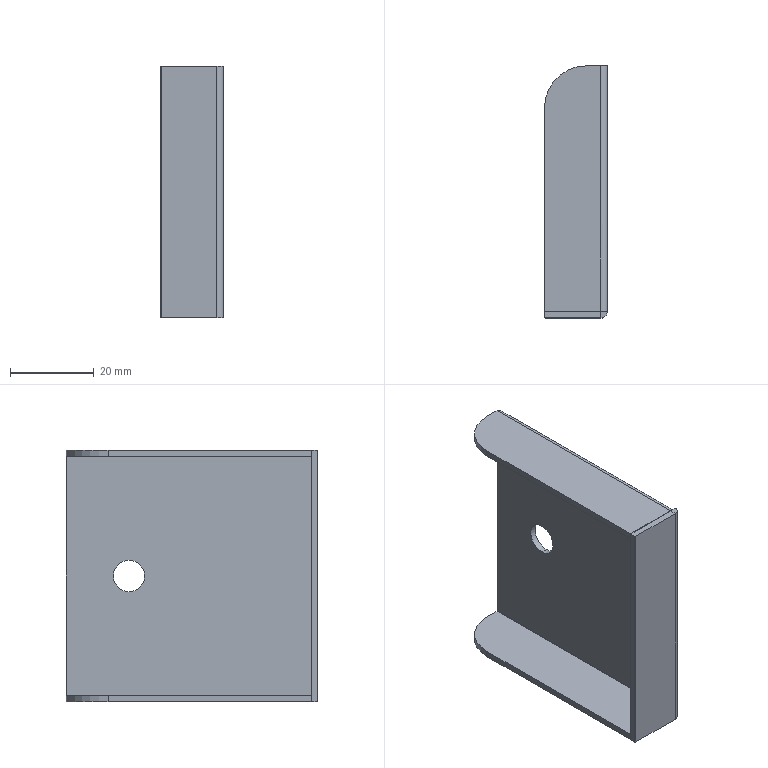Component | SolidWorks | BottomPlateWelding-2_AxisFixingPlate-2 | 1 solid | 37 faces | box 15 x 60 x 60 mm | volume 8752 mm3 | plane 27 | cylinder 10 | commonest cylinder face diameters 0.2 x3 3.2 x3 7.5 x2 20 x2
STEP:
#1=CARTESIAN_POINT('',(-9.252,0.7874,15.128));
#2=VERTEX_POINT('',#1);
#3=CARTESIAN_POINT('',(-9.252,0.7874,14.833));
#4=VERTEX_POINT('',#3);
#5=CARTESIAN_POINT('',(-9.252,0.7874,14.98));
#6=DIRECTION('',(1.,0.,-0.));
#7=DIRECTION('',(0.,0.,1.));
#8=AXIS2_PLACEMENT_3D('',#5,#6,#7);
#9=CIRCLE('',#8,0.1476);
#10=EDGE_CURVE('',#2,#4,#9,.T.);
#11=ORIENTED_EDGE('',*,*,#10,.F.);
#12=CARTESIAN_POINT('',(-9.193,0.7874,15.128));
#13=VERTEX_POINT('',#12);
#14=CARTESIAN_POINT('',(-9.67,0.7874,15.128));
#15=DIRECTION('',(1.,0.,-0.));
#16=VECTOR('',#15,39.37);
#17=LINE('',#14,#16);
#18=EDGE_CURVE('',#2,#13,#17,.T.);
#19=ORIENTED_EDGE('',*,*,#18,.T.);
#20=CARTESIAN_POINT('',(-9.193,0.7874,14.833));
#21=VERTEX_POINT('',#20);
#22=CARTESIAN_POINT('',(-9.193,0.7874,14.98));
#23=DIRECTION('',(1.,0.,-0.));
#24=DIRECTION('',(0.,-0.,-1.));
#25=AXIS2_PLACEMENT_3D('',#22,#23,#24);
#26=CIRCLE('',#25,0.1476);
#27=EDGE_CURVE('',#13,#21,#26,.T.);
#28=ORIENTED_EDGE('',*,*,#27,.T.);
#29=CARTESIAN_POINT('',(-9.67,0.7874,14.833));
#30=DIRECTION('',(1.,0.,-0.));
#31=VECTOR('',#30,39.37);
#32=LINE('',#29,#31);
#33=EDGE_CURVE('',#4,#21,#32,.T.);
#34=ORIENTED_EDGE('',*,*,#33,.F.);
#35=EDGE_LOOP('',(#11,#19,#28,#34));
#36=FACE_OUTER_BOUND('',#35,.T.);
#37=CARTESIAN_POINT('',(-9.67,0.7874,14.98));
#38=DIRECTION('',(1.,0.,-0.));
#39=DIRECTION('',(0.,-0.,-1.));
#40=AXIS2_PLACEMENT_3D('',#37,#38,#39);
#41=CYLINDRICAL_SURFACE('',#40,0.1476);
#42=ADVANCED_FACE('',(#36),#41,.F.);
#43=CARTESIAN_POINT('',(-9.193,-0.9213,16.161));
#44=VERTEX_POINT('',#43);
#45=CARTESIAN_POINT('',(-9.193,-0.9213,16.098));
#46=VERTEX_POINT('',#45);
#47=CARTESIAN_POINT('',(-9.193,-0.9213,13.799));
#48=DIRECTION('',(-0.,-0.,-1.));
#49=VECTOR('',#48,39.37);
#50=LINE('',#47,#49);
#51=EDGE_CURVE('',#44,#46,#50,.T.);
#52=ORIENTED_EDGE('',*,*,#51,.T.);
#53=CARTESIAN_POINT('',(-9.252,-0.9213,16.161));
#54=VERTEX_POINT('',#53);
#55=CARTESIAN_POINT('',(-9.256,-0.9213,16.098));
#56=DIRECTION('',(0.,-1.,0.));
#57=DIRECTION('',(0.,-0.,-1.));
#58=AXIS2_PLACEMENT_3D('',#55,#56,#57);
#59=CIRCLE('',#58,0.06299);
#60=EDGE_CURVE('',#46,#54,#59,.T.);
#61=ORIENTED_EDGE('',*,*,#60,.T.);
#62=CARTESIAN_POINT('',(-9.252,-0.9213,16.161));
#63=VERTEX_POINT('',#62);
#64=CARTESIAN_POINT('',(-9.252,-0.9213,16.098));
#65=DIRECTION('',(0.,0.,1.));
#66=VECTOR('',#65,39.37);
#67=LINE('',#64,#66);
#68=EDGE_CURVE('',#54,#63,#67,.T.);
#69=ORIENTED_EDGE('',*,*,#68,.T.);
#70=CARTESIAN_POINT('',(-9.252,-0.9213,16.161));
#71=DIRECTION('',(1.,-0.,-0.));
#72=VECTOR('',#71,39.37);
#73=LINE('',#70,#72);
#74=EDGE_CURVE('',#63,#44,#73,.T.);
#75=ORIENTED_EDGE('',*,*,#74,.T.);
#76=EDGE_LOOP('',(#52,#61,#69,#75));
#77=FACE_OUTER_BOUND('',#76,.T.);
#78=CARTESIAN_POINT('',(-9.252,-0.9213,16.098));
#79=DIRECTION('',(-0.,1.,-0.));
#80=DIRECTION('',(-0.,-0.,-1.));
#81=AXIS2_PLACEMENT_3D('',#78,#79,#80);
#82=PLANE('',#81);
#83=ADVANCED_FACE('',(#77),#82,.T.);
#84=CARTESIAN_POINT('',(-9.252,0.7874,14.98));
#85=DIRECTION('',(1.,0.,-0.));
#86=DIRECTION('',(0.,0.,1.));
#87=AXIS2_PLACEMENT_3D('',#84,#85,#86);
#88=CIRCLE('',#87,0.1476);
#89=EDGE_CURVE('',#4,#2,#88,.T.);
#90=ORIENTED_EDGE('',*,*,#89,.T.);
#91=ORIENTED_EDGE('',*,*,#10,.T.);
#92=EDGE_LOOP('',(#90,#91));
#93=FACE_BOUND('',#92,.T.);
#94=CARTESIAN_POINT('',(-9.252,-0.9213,13.862));
#95=VERTEX_POINT('',#94);
#96=CARTESIAN_POINT('',(-9.252,-0.9213,16.098));
#97=VERTEX_POINT('',#96);
#98=CARTESIAN_POINT('',(-9.252,-0.9213,13.799));
#99=DIRECTION('',(0.,0.,1.));
#100=VECTOR('',#99,39.37);
#101=LINE('',#98,#100);
#102=EDGE_CURVE('',#95,#97,#101,.T.);
#103=ORIENTED_EDGE('',*,*,#102,.T.);
#104=CARTESIAN_POINT('',(-9.252,1.378,16.098));
#105=VERTEX_POINT('',#104);
#106=CARTESIAN_POINT('',(-9.252,1.378,16.098));
#107=DIRECTION('',(0.,-1.,0.));
#108=VECTOR('',#107,39.37);
#109=LINE('',#106,#108);
#110=EDGE_CURVE('',#105,#97,#109,.T.);
#111=ORIENTED_EDGE('',*,*,#110,.F.);
#112=CARTESIAN_POINT('',(-9.252,1.378,13.862));
#113=VERTEX_POINT('',#112);
#114=CARTESIAN_POINT('',(-9.252,1.378,13.799));
#115=DIRECTION('',(0.,0.,1.));
#116=VECTOR('',#115,39.37);
#117=LINE('',#114,#116);
#118=EDGE_CURVE('',#113,#105,#117,.T.);
#119=ORIENTED_EDGE('',*,*,#118,.F.);
#120=CARTESIAN_POINT('',(-9.252,-0.9213,13.862));
#121=DIRECTION('',(-0.,1.,-0.));
#122=VECTOR('',#121,39.37);
#123=LINE('',#120,#122);
#124=EDGE_CURVE('',#95,#113,#123,.T.);
#125=ORIENTED_EDGE('',*,*,#124,.F.);
#126=EDGE_LOOP('',(#103,#111,#119,#125));
#127=FACE_OUTER_BOUND('',#126,.T.);
#128=CARTESIAN_POINT('',(-9.252,1.378,13.799));
#129=DIRECTION('',(-1.,-0.,0.));
#130=DIRECTION('',(0.,0.,1.));
#131=AXIS2_PLACEMENT_3D('',#128,#129,#130);
#132=PLANE('',#131);
#133=ADVANCED_FACE('',(#93,#127),#132,.T.);
#134=CARTESIAN_POINT('',(-9.193,0.7874,14.98));
#135=DIRECTION('',(1.,0.,-0.));
#136=DIRECTION('',(0.,-0.,-1.));
#137=AXIS2_PLACEMENT_3D('',#134,#135,#136);
#138=CIRCLE('',#137,0.1476);
#139=EDGE_CURVE('',#21,#13,#138,.T.);
#140=ORIENTED_EDGE('',*,*,#139,.F.);
#141=ORIENTED_EDGE('',*,*,#27,.F.);
#142=EDGE_LOOP('',(#140,#141));
#143=FACE_BOUND('',#142,.T.);
#144=CARTESIAN_POINT('',(-9.193,1.378,16.098));
#145=VERTEX_POINT('',#144);
#146=CARTESIAN_POINT('',(-9.193,1.378,16.098));
#147=DIRECTION('',(0.,-1.,0.));
#148=VECTOR('',#147,39.37);
#149=LINE('',#146,#148);
#150=EDGE_CURVE('',#145,#46,#149,.T.);
#151=ORIENTED_EDGE('',*,*,#150,.T.);
#152=CARTESIAN_POINT('',(-9.193,-0.9213,13.862));
#153=VERTEX_POINT('',#152);
#154=CARTESIAN_POINT('',(-9.193,-0.9213,13.799));
#155=DIRECTION('',(0.,0.,1.));
#156=VECTOR('',#155,39.37);
#157=LINE('',#154,#156);
#158=EDGE_CURVE('',#153,#46,#157,.T.);
#159=ORIENTED_EDGE('',*,*,#158,.F.);
#160=CARTESIAN_POINT('',(-9.193,1.378,13.862));
#161=VERTEX_POINT('',#160);
#162=CARTESIAN_POINT('',(-9.193,-0.9213,13.862));
#163=DIRECTION('',(-0.,1.,-0.));
#164=VECTOR('',#163,39.37);
#165=LINE('',#162,#164);
#166=EDGE_CURVE('',#153,#161,#165,.T.);
#167=ORIENTED_EDGE('',*,*,#166,.T.);
#168=CARTESIAN_POINT('',(-9.193,1.378,13.799));
#169=DIRECTION('',(0.,0.,1.));
#170=VECTOR('',#169,39.37);
#171=LINE('',#168,#170);
#172=EDGE_CURVE('',#161,#145,#171,.T.);
#173=ORIENTED_EDGE('',*,*,#172,.T.);
#174=EDGE_LOOP('',(#151,#159,#167,#173));
#175=FACE_OUTER_BOUND('',#174,.T.);
#176=CARTESIAN_POINT('',(-9.193,1.378,13.799));
#177=DIRECTION('',(-1.,-0.,0.));
#178=DIRECTION('',(0.,0.,1.));
#179=AXIS2_PLACEMENT_3D('',#176,#177,#178);
#180=PLANE('',#179);
#181=ADVANCED_FACE('',(#143,#175),#180,.F.);
#182=ORIENTED_EDGE('',*,*,#118,.T.);
#183=CARTESIAN_POINT('',(-9.252,1.378,16.098));
#184=DIRECTION('',(1.,0.,-0.));
#185=VECTOR('',#184,39.37);
#186=LINE('',#183,#185);
#187=EDGE_CURVE('',#105,#145,#186,.T.);
#188=ORIENTED_EDGE('',*,*,#187,.T.);
#189=ORIENTED_EDGE('',*,*,#172,.F.);
#190=CARTESIAN_POINT('',(-9.252,1.378,13.862));
#191=DIRECTION('',(1.,0.,-0.));
#192=VECTOR('',#191,39.37);
#193=LINE('',#190,#192);
#194=EDGE_CURVE('',#113,#161,#193,.T.);
#195=ORIENTED_EDGE('',*,*,#194,.F.);
#196=EDGE_LOOP('',(#182,#188,#189,#195));
#197=FACE_OUTER_BOUND('',#196,.T.);
#198=CARTESIAN_POINT('',(-9.193,1.378,13.799));
#199=DIRECTION('',(-0.,1.,-0.));
#200=DIRECTION('',(-0.,-0.,-1.));
#201=AXIS2_PLACEMENT_3D('',#198,#199,#200);
#202=PLANE('',#201);
#203=ADVANCED_FACE('',(#197),#202,.T.);
#204=CARTESIAN_POINT('',(-9.252,-0.9213,13.799));
#205=VERTEX_POINT('',#204);
#206=CARTESIAN_POINT('',(-9.252,-0.9213,13.799));
#207=VERTEX_POINT('',#206);
#208=CARTESIAN_POINT('',(-9.252,-0.9213,13.799));
#209=DIRECTION('',(0.,0.,1.));
#210=VECTOR('',#209,39.37);
#211=LINE('',#208,#210);
#212=EDGE_CURVE('',#205,#207,#211,.T.);
#213=ORIENTED_EDGE('',*,*,#212,.T.);
#214=CARTESIAN_POINT('',(-9.256,-0.9213,13.862));
#215=DIRECTION('',(0.,-1.,0.));
#216=DIRECTION('',(0.,0.,1.));
#217=AXIS2_PLACEMENT_3D('',#214,#215,#216);
#218=CIRCLE('',#217,0.06299);
#219=EDGE_CURVE('',#207,#153,#218,.T.);
#220=ORIENTED_EDGE('',*,*,#219,.T.);
#221=CARTESIAN_POINT('',(-9.193,-0.9213,13.799));
#222=VERTEX_POINT('',#221);
#223=CARTESIAN_POINT('',(-9.193,-0.9213,13.799));
#224=DIRECTION('',(0.,0.,1.));
#225=VECTOR('',#224,39.37);
#226=LINE('',#223,#225);
#227=EDGE_CURVE('',#222,#153,#226,.T.);
#228=ORIENTED_EDGE('',*,*,#227,.F.);
#229=CARTESIAN_POINT('',(-9.193,-0.9213,13.799));
#230=DIRECTION('',(-1.,0.,0.));
#231=VECTOR('',#230,39.37);
#232=LINE('',#229,#231);
#233=EDGE_CURVE('',#222,#205,#232,.T.);
#234=ORIENTED_EDGE('',*,*,#233,.T.);
#235=EDGE_LOOP('',(#213,#220,#228,#234));
#236=FACE_OUTER_BOUND('',#235,.T.);
#237=CARTESIAN_POINT('',(-9.252,-0.9213,13.799));
#238=DIRECTION('',(-0.,1.,-0.));
#239=DIRECTION('',(-0.,-0.,-1.));
#240=AXIS2_PLACEMENT_3D('',#237,#238,#239);
#241=PLANE('',#240);
#242=ADVANCED_FACE('',(#236),#241,.T.);
#243=ORIENTED_EDGE('',*,*,#233,.F.);
#244=CARTESIAN_POINT('',(-9.256,-0.9843,13.799));
#245=VERTEX_POINT('',#244);
#246=CARTESIAN_POINT('',(-9.256,-0.9213,13.799));
#247=DIRECTION('',(-0.,-0.,-1.));
#248=DIRECTION('',(1.,0.,0.));
#249=AXIS2_PLACEMENT_3D('',#246,#247,#248);
#250=CIRCLE('',#249,0.06299);
#251=EDGE_CURVE('',#222,#245,#250,.T.);
#252=ORIENTED_EDGE('',*,*,#251,.T.);
#253=CARTESIAN_POINT('',(-9.256,-0.9252,13.799));
#254=VERTEX_POINT('',#253);
#255=CARTESIAN_POINT('',(-9.256,-0.9252,13.799));
#256=DIRECTION('',(0.,-1.,0.));
#257=VECTOR('',#256,39.37);
#258=LINE('',#255,#257);
#259=EDGE_CURVE('',#254,#245,#258,.T.);
#260=ORIENTED_EDGE('',*,*,#259,.F.);
#261=CARTESIAN_POINT('',(-9.256,-0.9213,13.799));
#262=DIRECTION('',(-0.,-0.,-1.));
#263=DIRECTION('',(-1.,0.,0.));
#264=AXIS2_PLACEMENT_3D('',#261,#262,#263);
#265=CIRCLE('',#264,0.003937);
#266=EDGE_CURVE('',#205,#254,#265,.T.);
#267=ORIENTED_EDGE('',*,*,#266,.F.);
#268=EDGE_LOOP('',(#243,#252,#260,#267));
#269=FACE_OUTER_BOUND('',#268,.T.);
#270=CARTESIAN_POINT('',(-9.193,-0.9213,13.799));
#271=DIRECTION('',(-0.,-0.,-1.));
#272=DIRECTION('',(-1.,-0.,0.));
#273=AXIS2_PLACEMENT_3D('',#270,#271,#272);
#274=PLANE('',#273);
#275=ADVANCED_FACE('',(#269),#274,.T.);
#276=CARTESIAN_POINT('',(-9.256,-0.9843,16.161));
#277=VERTEX_POINT('',#276);
#278=CARTESIAN_POINT('',(-9.256,-0.9252,16.161));
#279=VERTEX_POINT('',#278);
#280=CARTESIAN_POINT('',(-9.256,-0.9843,16.161));
#281=DIRECTION('',(-0.,1.,-0.));
#282=VECTOR('',#281,39.37);
#283=LINE('',#280,#282);
#284=EDGE_CURVE('',#277,#279,#283,.T.);
#285=ORIENTED_EDGE('',*,*,#284,.F.);
#286=CARTESIAN_POINT('',(-9.256,-0.9213,16.161));
#287=DIRECTION('',(-0.,-0.,-1.));
#288=DIRECTION('',(1.,0.,0.));
#289=AXIS2_PLACEMENT_3D('',#286,#287,#288);
#290=CIRCLE('',#289,0.06299);
#291=EDGE_CURVE('',#44,#277,#290,.T.);
#292=ORIENTED_EDGE('',*,*,#291,.F.);
#293=ORIENTED_EDGE('',*,*,#74,.F.);
#294=CARTESIAN_POINT('',(-9.256,-0.9213,16.161));
#295=DIRECTION('',(-0.,-0.,-1.));
#296=DIRECTION('',(-1.,0.,0.));
#297=AXIS2_PLACEMENT_3D('',#294,#295,#296);
#298=CIRCLE('',#297,0.003937);
#299=EDGE_CURVE('',#63,#279,#298,.T.);
#300=ORIENTED_EDGE('',*,*,#299,.T.);
#301=EDGE_LOOP('',(#285,#292,#293,#300));
#302=FACE_OUTER_BOUND('',#301,.T.);
#303=CARTESIAN_POINT('',(-9.256,-0.9843,16.161));
#304=DIRECTION('',(0.,0.,1.));
#305=DIRECTION('',(1.,0.,-0.));
#306=AXIS2_PLACEMENT_3D('',#303,#304,#305);
#307=PLANE('',#306);
#308=ADVANCED_FACE('',(#302),#307,.T.);
#309=CARTESIAN_POINT('',(-9.783,-0.9252,16.161));
#310=VERTEX_POINT('',#309);
#311=CARTESIAN_POINT('',(-9.783,-0.9783,16.161));
#312=VERTEX_POINT('',#311);
#313=CARTESIAN_POINT('',(-9.783,-0.9252,16.161));
#314=DIRECTION('',(0.,-1.,0.));
#315=VECTOR('',#314,39.37);
#316=LINE('',#313,#315);
#317=EDGE_CURVE('',#310,#312,#316,.T.);
#318=ORIENTED_EDGE('',*,*,#317,.T.);
#319=CARTESIAN_POINT('',(-9.778,-0.9843,16.161));
#320=VERTEX_POINT('',#319);
#321=CARTESIAN_POINT('',(-9.546,-1.216,16.161));
#322=DIRECTION('',(0.7071,-0.7071,0.));
#323=VECTOR('',#322,39.37);
#324=LINE('',#321,#323);
#325=EDGE_CURVE('',#312,#320,#324,.T.);
#326=ORIENTED_EDGE('',*,*,#325,.T.);
#327=CARTESIAN_POINT('',(-9.193,-0.9843,16.161));
#328=DIRECTION('',(-1.,-0.,0.));
#329=VECTOR('',#328,39.37);
#330=LINE('',#327,#329);
#331=EDGE_CURVE('',#277,#320,#330,.T.);
#332=ORIENTED_EDGE('',*,*,#331,.F.);
#333=ORIENTED_EDGE('',*,*,#284,.T.);
#334=CARTESIAN_POINT('',(-9.193,-0.9252,16.161));
#335=DIRECTION('',(-1.,-0.,0.));
#336=VECTOR('',#335,39.37);
#337=LINE('',#334,#336);
#338=EDGE_CURVE('',#279,#310,#337,.T.);
#339=ORIENTED_EDGE('',*,*,#338,.T.);
#340=EDGE_LOOP('',(#318,#326,#332,#333,#339));
#341=FACE_OUTER_BOUND('',#340,.T.);
#342=CARTESIAN_POINT('',(-9.252,-0.9213,16.161));
#343=DIRECTION('',(0.,0.,1.));
#344=DIRECTION('',(1.,0.,-0.));
#345=AXIS2_PLACEMENT_3D('',#342,#343,#344);
#346=PLANE('',#345);
#347=ADVANCED_FACE('',(#341),#346,.T.);
#348=ORIENTED_EDGE('',*,*,#331,.T.);
#349=CARTESIAN_POINT('',(-9.778,-0.9843,13.799));
#350=VERTEX_POINT('',#349);
#351=CARTESIAN_POINT('',(-9.778,-0.9843,13.799));
#352=DIRECTION('',(-0.,-0.,-1.));
#353=VECTOR('',#352,39.37);
#354=LINE('',#351,#353);
#355=EDGE_CURVE('',#320,#350,#354,.T.);
#356=ORIENTED_EDGE('',*,*,#355,.T.);
#357=CARTESIAN_POINT('',(-9.193,-0.9843,13.799));
#358=DIRECTION('',(-1.,-0.,0.));
#359=VECTOR('',#358,39.37);
#360=LINE('',#357,#359);
#361=EDGE_CURVE('',#245,#350,#360,.T.);
#362=ORIENTED_EDGE('',*,*,#361,.F.);
#363=CARTESIAN_POINT('',(-9.256,-0.9843,13.799));
#364=DIRECTION('',(0.,0.,1.));
#365=VECTOR('',#364,39.37);
#366=LINE('',#363,#365);
#367=EDGE_CURVE('',#245,#277,#366,.T.);
#368=ORIENTED_EDGE('',*,*,#367,.T.);
#369=EDGE_LOOP('',(#348,#356,#362,#368));
#370=FACE_OUTER_BOUND('',#369,.T.);
#371=CARTESIAN_POINT('',(-9.193,-0.9843,13.799));
#372=DIRECTION('',(-0.,1.,-0.));
#373=DIRECTION('',(-0.,-0.,-1.));
#374=AXIS2_PLACEMENT_3D('',#371,#372,#373);
#375=PLANE('',#374);
#376=ADVANCED_FACE('',(#370),#375,.F.);
#377=CARTESIAN_POINT('',(-9.783,-0.9252,13.799));
#378=VERTEX_POINT('',#377);
#379=CARTESIAN_POINT('',(-9.783,-0.9783,13.799));
#380=VERTEX_POINT('',#379);
#381=CARTESIAN_POINT('',(-9.783,-0.9252,13.799));
#382=DIRECTION('',(0.,-1.,0.));
#383=VECTOR('',#382,39.37);
#384=LINE('',#381,#383);
#385=EDGE_CURVE('',#378,#380,#384,.T.);
#386=ORIENTED_EDGE('',*,*,#385,.T.);
#387=CARTESIAN_POINT('',(-9.783,-0.9783,16.161));
#388=DIRECTION('',(0.,0.,1.));
#389=VECTOR('',#388,39.37);
#390=LINE('',#387,#389);
#391=EDGE_CURVE('',#380,#312,#390,.T.);
#392=ORIENTED_EDGE('',*,*,#391,.T.);
#393=ORIENTED_EDGE('',*,*,#317,.F.);
#394=CARTESIAN_POINT('',(-9.783,-0.9252,13.799));
#395=DIRECTION('',(0.,0.,1.));
#396=VECTOR('',#395,39.37);
#397=LINE('',#394,#396);
#398=EDGE_CURVE('',#378,#310,#397,.T.);
#399=ORIENTED_EDGE('',*,*,#398,.F.);
#400=EDGE_LOOP('',(#386,#392,#393,#399));
#401=FACE_OUTER_BOUND('',#400,.T.);
#402=CARTESIAN_POINT('',(-9.783,-0.9252,13.799));
#403=DIRECTION('',(-1.,-0.,0.));
#404=DIRECTION('',(0.,0.,1.));
#405=AXIS2_PLACEMENT_3D('',#402,#403,#404);
#406=PLANE('',#405);
#407=ADVANCED_FACE('',(#401),#406,.T.);
#408=ORIENTED_EDGE('',*,*,#338,.F.);
#409=CARTESIAN_POINT('',(-9.256,-0.9252,13.799));
#410=DIRECTION('',(0.,0.,1.));
#411=VECTOR('',#410,39.37);
#412=LINE('',#409,#411);
#413=EDGE_CURVE('',#254,#279,#412,.T.);
#414=ORIENTED_EDGE('',*,*,#413,.F.);
#415=CARTESIAN_POINT('',(-9.193,-0.9252,13.799));
#416=DIRECTION('',(-1.,-0.,0.));
#417=VECTOR('',#416,39.37);
#418=LINE('',#415,#417);
#419=EDGE_CURVE('',#254,#378,#418,.T.);
#420=ORIENTED_EDGE('',*,*,#419,.T.);
#421=ORIENTED_EDGE('',*,*,#398,.T.);
#422=EDGE_LOOP('',(#408,#414,#420,#421));
#423=FACE_OUTER_BOUND('',#422,.T.);
#424=CARTESIAN_POINT('',(-9.193,-0.9252,13.799));
#425=DIRECTION('',(-0.,1.,-0.));
#426=DIRECTION('',(-0.,-0.,-1.));
#427=AXIS2_PLACEMENT_3D('',#424,#425,#426);
#428=PLANE('',#427);
#429=ADVANCED_FACE('',(#423),#428,.T.);
#430=ORIENTED_EDGE('',*,*,#299,.F.);
#431=ORIENTED_EDGE('',*,*,#68,.F.);
#432=CARTESIAN_POINT('',(-9.252,-0.9213,16.098));
#433=DIRECTION('',(0.,0.,1.));
#434=VECTOR('',#433,39.37);
#435=LINE('',#432,#434);
#436=EDGE_CURVE('',#97,#54,#435,.T.);
#437=ORIENTED_EDGE('',*,*,#436,.F.);
#438=ORIENTED_EDGE('',*,*,#102,.F.);
#439=CARTESIAN_POINT('',(-9.252,-0.9213,13.799));
#440=DIRECTION('',(0.,0.,1.));
#441=VECTOR('',#440,39.37);
#442=LINE('',#439,#441);
#443=EDGE_CURVE('',#207,#95,#442,.T.);
#444=ORIENTED_EDGE('',*,*,#443,.F.);
#445=ORIENTED_EDGE('',*,*,#212,.F.);
#446=ORIENTED_EDGE('',*,*,#266,.T.);
#447=ORIENTED_EDGE('',*,*,#413,.T.);
#448=EDGE_LOOP('',(#430,#431,#437,#438,#444,#445,#446,#447));
#449=FACE_OUTER_BOUND('',#448,.T.);
#450=CARTESIAN_POINT('',(-9.256,-0.9213,13.799));
#451=DIRECTION('',(0.,0.,1.));
#452=DIRECTION('',(1.,0.,0.));
#453=AXIS2_PLACEMENT_3D('',#450,#451,#452);
#454=CYLINDRICAL_SURFACE('',#453,0.003937);
#455=ADVANCED_FACE('',(#449),#454,.F.);
#456=ORIENTED_EDGE('',*,*,#291,.T.);
#457=ORIENTED_EDGE('',*,*,#367,.F.);
#458=ORIENTED_EDGE('',*,*,#251,.F.);
#459=ORIENTED_EDGE('',*,*,#227,.T.);
#460=ORIENTED_EDGE('',*,*,#158,.T.);
#461=ORIENTED_EDGE('',*,*,#51,.F.);
#462=EDGE_LOOP('',(#456,#457,#458,#459,#460,#461));
#463=FACE_OUTER_BOUND('',#462,.T.);
#464=CARTESIAN_POINT('',(-9.256,-0.9213,13.799));
#465=DIRECTION('',(0.,0.,1.));
#466=DIRECTION('',(1.,0.,0.));
#467=AXIS2_PLACEMENT_3D('',#464,#465,#466);
#468=CYLINDRICAL_SURFACE('',#467,0.06299);
#469=ADVANCED_FACE('',(#463),#468,.T.);
#470=ORIENTED_EDGE('',*,*,#361,.T.);
#471=CARTESIAN_POINT('',(-9.548,-1.214,13.799));
#472=DIRECTION('',(-0.7071,0.7071,-0.));
#473=VECTOR('',#472,39.37);
#474=LINE('',#471,#473);
#475=EDGE_CURVE('',#350,#380,#474,.T.);
#476=ORIENTED_EDGE('',*,*,#475,.T.);
#477=ORIENTED_EDGE('',*,*,#385,.F.);
#478=ORIENTED_EDGE('',*,*,#419,.F.);
#479=ORIENTED_EDGE('',*,*,#259,.T.);
#480=EDGE_LOOP('',(#470,#476,#477,#478,#479));
#481=FACE_OUTER_BOUND('',#480,.T.);
#482=CARTESIAN_POINT('',(-9.256,-0.9213,13.799));
#483=DIRECTION('',(-0.,-0.,-1.));
#484=DIRECTION('',(-1.,-0.,0.));
#485=AXIS2_PLACEMENT_3D('',#482,#483,#484);
#486=PLANE('',#485);
#487=ADVANCED_FACE('',(#481),#486,.T.);
#488=ORIENTED_EDGE('',*,*,#18,.F.);
#489=ORIENTED_EDGE('',*,*,#89,.F.);
#490=ORIENTED_EDGE('',*,*,#33,.T.);
#491=ORIENTED_EDGE('',*,*,#139,.T.);
#492=EDGE_LOOP('',(#488,#489,#490,#491));
#493=FACE_OUTER_BOUND('',#492,.T.);
#494=CARTESIAN_POINT('',(-9.67,0.7874,14.98));
#495=DIRECTION('',(1.,0.,-0.));
#496=DIRECTION('',(0.,-0.,-1.));
#497=AXIS2_PLACEMENT_3D('',#494,#495,#496);
#498=CYLINDRICAL_SURFACE('',#497,0.1476);
#499=ADVANCED_FACE('',(#493),#498,.F.);
#500=CARTESIAN_POINT('',(-9.256,1.378,13.858));
#501=VERTEX_POINT('',#500);
#502=CARTESIAN_POINT('',(-9.256,1.378,13.799));
#503=VERTEX_POINT('',#502);
#504=CARTESIAN_POINT('',(-9.256,1.378,13.799));
#505=DIRECTION('',(-0.,-0.,-1.));
#506=VECTOR('',#505,39.37);
#507=LINE('',#504,#506);
#508=EDGE_CURVE('',#501,#503,#507,.T.);
#509=ORIENTED_EDGE('',*,*,#508,.F.);
#510=CARTESIAN_POINT('',(-9.256,1.378,13.862));
#511=DIRECTION('',(-0.,1.,-0.));
#512=DIRECTION('',(0.,0.,1.));
#513=AXIS2_PLACEMENT_3D('',#510,#511,#512);
#514=CIRCLE('',#513,0.003937);
#515=EDGE_CURVE('',#113,#501,#514,.T.);
#516=ORIENTED_EDGE('',*,*,#515,.F.);
#517=ORIENTED_EDGE('',*,*,#194,.T.);
#518=CARTESIAN_POINT('',(-9.256,1.378,13.862));
#519=DIRECTION('',(-0.,1.,-0.));
#520=DIRECTION('',(0.,0.,1.));
#521=AXIS2_PLACEMENT_3D('',#518,#519,#520);
#522=CIRCLE('',#521,0.06299);
#523=EDGE_CURVE('',#161,#503,#522,.T.);
#524=ORIENTED_EDGE('',*,*,#523,.T.);
#525=EDGE_LOOP('',(#509,#516,#517,#524));
#526=FACE_OUTER_BOUND('',#525,.T.);
#527=CARTESIAN_POINT('',(-9.256,1.378,13.862));
#528=DIRECTION('',(-0.,1.,-0.));
#529=DIRECTION('',(-0.,-0.,-1.));
#530=AXIS2_PLACEMENT_3D('',#527,#528,#529);
#531=PLANE('',#530);
#532=ADVANCED_FACE('',(#526),#531,.T.);
#533=CARTESIAN_POINT('',(-9.256,-0.9213,13.799));
#534=VERTEX_POINT('',#533);
#535=CARTESIAN_POINT('',(-9.256,-0.9213,13.862));
#536=DIRECTION('',(0.,-1.,0.));
#537=DIRECTION('',(0.,0.,1.));
#538=AXIS2_PLACEMENT_3D('',#535,#536,#537);
#539=CIRCLE('',#538,0.06299);
#540=EDGE_CURVE('',#534,#207,#539,.T.);
#541=ORIENTED_EDGE('',*,*,#540,.T.);
#542=ORIENTED_EDGE('',*,*,#443,.T.);
#543=CARTESIAN_POINT('',(-9.256,-0.9213,13.858));
#544=VERTEX_POINT('',#543);
#545=CARTESIAN_POINT('',(-9.256,-0.9213,13.862));
#546=DIRECTION('',(0.,-1.,0.));
#547=DIRECTION('',(0.,0.,1.));
#548=AXIS2_PLACEMENT_3D('',#545,#546,#547);
#549=CIRCLE('',#548,0.003937);
#550=EDGE_CURVE('',#544,#95,#549,.T.);
#551=ORIENTED_EDGE('',*,*,#550,.F.);
#552=CARTESIAN_POINT('',(-9.256,-0.9213,13.858));
#553=DIRECTION('',(-0.,-0.,-1.));
#554=VECTOR('',#553,39.37);
#555=LINE('',#552,#554);
#556=EDGE_CURVE('',#544,#534,#555,.T.);
#557=ORIENTED_EDGE('',*,*,#556,.T.);
#558=EDGE_LOOP('',(#541,#542,#551,#557));
#559=FACE_OUTER_BOUND('',#558,.T.);
#560=CARTESIAN_POINT('',(-9.256,-0.9213,13.862));
#561=DIRECTION('',(-0.,1.,-0.));
#562=DIRECTION('',(-0.,-0.,-1.));
#563=AXIS2_PLACEMENT_3D('',#560,#561,#562);
#564=PLANE('',#563);
#565=ADVANCED_FACE('',(#559),#564,.F.);
#566=ORIENTED_EDGE('',*,*,#166,.F.);
#567=ORIENTED_EDGE('',*,*,#219,.F.);
#568=ORIENTED_EDGE('',*,*,#540,.F.);
#569=CARTESIAN_POINT('',(-9.256,-0.9843,13.799));
#570=DIRECTION('',(0.,-1.,0.));
#571=VECTOR('',#570,39.37);
#572=LINE('',#569,#571);
#573=EDGE_CURVE('',#503,#534,#572,.T.);
#574=ORIENTED_EDGE('',*,*,#573,.F.);
#575=ORIENTED_EDGE('',*,*,#523,.F.);
#576=EDGE_LOOP('',(#566,#567,#568,#574,#575));
#577=FACE_OUTER_BOUND('',#576,.T.);
#578=CARTESIAN_POINT('',(-9.256,-0.9213,13.862));
#579=DIRECTION('',(0.,-1.,0.));
#580=DIRECTION('',(0.,-0.,-1.));
#581=AXIS2_PLACEMENT_3D('',#578,#579,#580);
#582=CYLINDRICAL_SURFACE('',#581,0.06299);
#583=ADVANCED_FACE('',(#577),#582,.T.);
#584=ORIENTED_EDGE('',*,*,#124,.T.);
#585=ORIENTED_EDGE('',*,*,#515,.T.);
#586=CARTESIAN_POINT('',(-9.256,1.378,13.858));
#587=DIRECTION('',(0.,-1.,0.));
#588=VECTOR('',#587,39.37);
#589=LINE('',#586,#588);
#590=EDGE_CURVE('',#501,#544,#589,.T.);
#591=ORIENTED_EDGE('',*,*,#590,.T.);
#592=ORIENTED_EDGE('',*,*,#550,.T.);
#593=EDGE_LOOP('',(#584,#585,#591,#592));
#594=FACE_OUTER_BOUND('',#593,.T.);
#595=CARTESIAN_POINT('',(-9.256,-0.9213,13.862));
#596=DIRECTION('',(0.,-1.,0.));
#597=DIRECTION('',(0.,0.,-1.));
#598=AXIS2_PLACEMENT_3D('',#595,#596,#597);
#599=CYLINDRICAL_SURFACE('',#598,0.003937);
#600=ADVANCED_FACE('',(#594),#599,.F.);
#601=CARTESIAN_POINT('',(-9.39,1.378,13.799));
#602=VERTEX_POINT('',#601);
#603=CARTESIAN_POINT('',(-9.193,1.378,13.799));
#604=DIRECTION('',(1.,0.,0.));
#605=VECTOR('',#604,39.37);
#606=LINE('',#603,#605);
#607=EDGE_CURVE('',#602,#503,#606,.T.);
#608=ORIENTED_EDGE('',*,*,#607,.F.);
#609=CARTESIAN_POINT('',(-9.39,1.378,13.858));
#610=VERTEX_POINT('',#609);
#611=CARTESIAN_POINT('',(-9.39,1.378,13.799));
#612=DIRECTION('',(-0.,0.,1.));
#613=VECTOR('',#612,39.37);
#614=LINE('',#611,#613);
#615=EDGE_CURVE('',#602,#610,#614,.T.);
#616=ORIENTED_EDGE('',*,*,#615,.T.);
#617=CARTESIAN_POINT('',(-9.252,1.378,13.858));
#618=DIRECTION('',(1.,0.,0.));
#619=VECTOR('',#618,39.37);
#620=LINE('',#617,#619);
#621=EDGE_CURVE('',#610,#501,#620,.T.);
#622=ORIENTED_EDGE('',*,*,#621,.T.);
#623=ORIENTED_EDGE('',*,*,#508,.T.);
#624=EDGE_LOOP('',(#608,#616,#622,#623));
#625=FACE_OUTER_BOUND('',#624,.T.);
#626=CARTESIAN_POINT('',(-9.252,1.378,13.799));
#627=DIRECTION('',(0.,-1.,0.));
#628=DIRECTION('',(0.,0.,1.));
#629=AXIS2_PLACEMENT_3D('',#626,#627,#628);
#630=PLANE('',#629);
#631=ADVANCED_FACE('',(#625),#630,.F.);
#632=ORIENTED_EDGE('',*,*,#556,.F.);
#633=CARTESIAN_POINT('',(-9.783,-0.9213,13.858));
#634=VERTEX_POINT('',#633);
#635=CARTESIAN_POINT('',(-9.783,-0.9213,13.858));
#636=DIRECTION('',(-1.,-0.,-0.));
#637=VECTOR('',#636,39.37);
#638=LINE('',#635,#637);
#639=EDGE_CURVE('',#544,#634,#638,.T.);
#640=ORIENTED_EDGE('',*,*,#639,.T.);
#641=CARTESIAN_POINT('',(-9.783,-0.9213,13.799));
#642=VERTEX_POINT('',#641);
#643=CARTESIAN_POINT('',(-9.783,-0.9213,13.799));
#644=DIRECTION('',(-0.,0.,1.));
#645=VECTOR('',#644,39.37);
#646=LINE('',#643,#645);
#647=EDGE_CURVE('',#642,#634,#646,.T.);
#648=ORIENTED_EDGE('',*,*,#647,.F.);
#649=CARTESIAN_POINT('',(-9.193,-0.9213,13.799));
#650=DIRECTION('',(-1.,-0.,-0.));
#651=VECTOR('',#650,39.37);
#652=LINE('',#649,#651);
#653=EDGE_CURVE('',#534,#642,#652,.T.);
#654=ORIENTED_EDGE('',*,*,#653,.F.);
#655=EDGE_LOOP('',(#632,#640,#648,#654));
#656=FACE_OUTER_BOUND('',#655,.T.);
#657=CARTESIAN_POINT('',(-9.783,-0.9213,13.799));
#658=DIRECTION('',(-0.,1.,-0.));
#659=DIRECTION('',(-0.,-0.,-1.));
#660=AXIS2_PLACEMENT_3D('',#657,#658,#659);
#661=PLANE('',#660);
#662=ADVANCED_FACE('',(#656),#661,.F.);
#663=CARTESIAN_POINT('',(-9.783,0.9843,13.799));
#664=VERTEX_POINT('',#663);
#665=CARTESIAN_POINT('',(-9.783,-0.9843,13.799));
#666=DIRECTION('',(-0.,1.,-0.));
#667=VECTOR('',#666,39.37);
#668=LINE('',#665,#667);
#669=EDGE_CURVE('',#642,#664,#668,.T.);
#670=ORIENTED_EDGE('',*,*,#669,.T.);
#671=CARTESIAN_POINT('',(-9.39,0.9843,13.799));
#672=DIRECTION('',(0.,-0.,-1.));
#673=DIRECTION('',(-1.,0.,0.));
#674=AXIS2_PLACEMENT_3D('',#671,#672,#673);
#675=CIRCLE('',#674,0.3937);
#676=EDGE_CURVE('',#664,#602,#675,.T.);
#677=ORIENTED_EDGE('',*,*,#676,.T.);
#678=ORIENTED_EDGE('',*,*,#607,.T.);
#679=ORIENTED_EDGE('',*,*,#573,.T.);
#680=ORIENTED_EDGE('',*,*,#653,.T.);
#681=EDGE_LOOP('',(#670,#677,#678,#679,#680));
#682=FACE_OUTER_BOUND('',#681,.T.);
#683=CARTESIAN_POINT('',(-9.193,-0.9843,13.799));
#684=DIRECTION('',(0.,-0.,-1.));
#685=DIRECTION('',(-1.,-0.,-0.));
#686=AXIS2_PLACEMENT_3D('',#683,#684,#685);
#687=PLANE('',#686);
#688=ADVANCED_FACE('',(#682),#687,.T.);
#689=ORIENTED_EDGE('',*,*,#621,.F.);
#690=CARTESIAN_POINT('',(-9.783,0.9843,13.858));
#691=VERTEX_POINT('',#690);
#692=CARTESIAN_POINT('',(-9.39,0.9843,13.858));
#693=DIRECTION('',(-0.,0.,1.));
#694=DIRECTION('',(-1.,0.,0.));
#695=AXIS2_PLACEMENT_3D('',#692,#693,#694);
#696=CIRCLE('',#695,0.3937);
#697=EDGE_CURVE('',#610,#691,#696,.T.);
#698=ORIENTED_EDGE('',*,*,#697,.T.);
#699=CARTESIAN_POINT('',(-9.783,-0.9213,13.858));
#700=DIRECTION('',(-0.,1.,-0.));
#701=VECTOR('',#700,39.37);
#702=LINE('',#699,#701);
#703=EDGE_CURVE('',#634,#691,#702,.T.);
#704=ORIENTED_EDGE('',*,*,#703,.F.);
#705=ORIENTED_EDGE('',*,*,#639,.F.);
#706=ORIENTED_EDGE('',*,*,#590,.F.);
#707=EDGE_LOOP('',(#689,#698,#704,#705,#706));
#708=FACE_OUTER_BOUND('',#707,.T.);
#709=CARTESIAN_POINT('',(-9.193,-0.9843,13.858));
#710=DIRECTION('',(0.,-0.,-1.));
#711=DIRECTION('',(-1.,-0.,-0.));
#712=AXIS2_PLACEMENT_3D('',#709,#710,#711);
#713=PLANE('',#712);
#714=ADVANCED_FACE('',(#708),#713,.F.);
#715=ORIENTED_EDGE('',*,*,#703,.T.);
#716=CARTESIAN_POINT('',(-9.783,0.9843,13.799));
#717=DIRECTION('',(0.,-0.,-1.));
#718=VECTOR('',#717,39.37);
#719=LINE('',#716,#718);
#720=EDGE_CURVE('',#691,#664,#719,.T.);
#721=ORIENTED_EDGE('',*,*,#720,.T.);
#722=ORIENTED_EDGE('',*,*,#669,.F.);
#723=ORIENTED_EDGE('',*,*,#647,.T.);
#724=EDGE_LOOP('',(#715,#721,#722,#723));
#725=FACE_OUTER_BOUND('',#724,.T.);
#726=CARTESIAN_POINT('',(-9.783,-0.9213,13.799));
#727=DIRECTION('',(1.,0.,0.));
#728=DIRECTION('',(0.,-0.,-1.));
#729=AXIS2_PLACEMENT_3D('',#726,#727,#728);
#730=PLANE('',#729);
#731=ADVANCED_FACE('',(#725),#730,.F.);
#732=CARTESIAN_POINT('',(-9.256,-0.9213,16.102));
#733=VERTEX_POINT('',#732);
#734=CARTESIAN_POINT('',(-9.256,-0.9213,16.098));
#735=DIRECTION('',(0.,-1.,0.));
#736=DIRECTION('',(0.,0.,-1.));
#737=AXIS2_PLACEMENT_3D('',#734,#735,#736);
#738=CIRCLE('',#737,0.003937);
#739=EDGE_CURVE('',#97,#733,#738,.T.);
#740=ORIENTED_EDGE('',*,*,#739,.F.);
#741=ORIENTED_EDGE('',*,*,#436,.T.);
#742=CARTESIAN_POINT('',(-9.256,-0.9213,16.161));
#743=VERTEX_POINT('',#742);
#744=CARTESIAN_POINT('',(-9.256,-0.9213,16.098));
#745=DIRECTION('',(0.,-1.,0.));
#746=DIRECTION('',(0.,-0.,-1.));
#747=AXIS2_PLACEMENT_3D('',#744,#745,#746);
#748=CIRCLE('',#747,0.06299);
#749=EDGE_CURVE('',#54,#743,#748,.T.);
#750=ORIENTED_EDGE('',*,*,#749,.T.);
#751=CARTESIAN_POINT('',(-9.256,-0.9213,16.161));
#752=DIRECTION('',(0.,0.,1.));
#753=VECTOR('',#752,39.37);
#754=LINE('',#751,#753);
#755=EDGE_CURVE('',#733,#743,#754,.T.);
#756=ORIENTED_EDGE('',*,*,#755,.F.);
#757=EDGE_LOOP('',(#740,#741,#750,#756));
#758=FACE_OUTER_BOUND('',#757,.T.);
#759=CARTESIAN_POINT('',(-9.256,-0.9213,16.098));
#760=DIRECTION('',(0.,-1.,0.));
#761=DIRECTION('',(0.,0.,1.));
#762=AXIS2_PLACEMENT_3D('',#759,#760,#761);
#763=PLANE('',#762);
#764=ADVANCED_FACE('',(#758),#763,.T.);
#765=CARTESIAN_POINT('',(-9.256,1.378,16.102));
#766=VERTEX_POINT('',#765);
#767=CARTESIAN_POINT('',(-9.256,1.378,16.098));
#768=DIRECTION('',(-0.,1.,-0.));
#769=DIRECTION('',(0.,0.,-1.));
#770=AXIS2_PLACEMENT_3D('',#767,#768,#769);
#771=CIRCLE('',#770,0.003937);
#772=EDGE_CURVE('',#766,#105,#771,.T.);
#773=ORIENTED_EDGE('',*,*,#772,.F.);
#774=CARTESIAN_POINT('',(-9.256,1.378,16.161));
#775=VERTEX_POINT('',#774);
#776=CARTESIAN_POINT('',(-9.256,1.378,16.102));
#777=DIRECTION('',(0.,0.,1.));
#778=VECTOR('',#777,39.37);
#779=LINE('',#776,#778);
#780=EDGE_CURVE('',#766,#775,#779,.T.);
#781=ORIENTED_EDGE('',*,*,#780,.T.);
#782=CARTESIAN_POINT('',(-9.256,1.378,16.098));
#783=DIRECTION('',(-0.,1.,-0.));
#784=DIRECTION('',(0.,-0.,-1.));
#785=AXIS2_PLACEMENT_3D('',#782,#783,#784);
#786=CIRCLE('',#785,0.06299);
#787=EDGE_CURVE('',#775,#145,#786,.T.);
#788=ORIENTED_EDGE('',*,*,#787,.T.);
#789=ORIENTED_EDGE('',*,*,#187,.F.);
#790=EDGE_LOOP('',(#773,#781,#788,#789));
#791=FACE_OUTER_BOUND('',#790,.T.);
#792=CARTESIAN_POINT('',(-9.256,1.378,16.098));
#793=DIRECTION('',(0.,-1.,0.));
#794=DIRECTION('',(0.,0.,1.));
#795=AXIS2_PLACEMENT_3D('',#792,#793,#794);
#796=PLANE('',#795);
#797=ADVANCED_FACE('',(#791),#796,.F.);
#798=ORIENTED_EDGE('',*,*,#150,.F.);
#799=ORIENTED_EDGE('',*,*,#787,.F.);
#800=CARTESIAN_POINT('',(-9.256,-0.9213,16.161));
#801=DIRECTION('',(0.,-1.,0.));
#802=VECTOR('',#801,39.37);
#803=LINE('',#800,#802);
#804=EDGE_CURVE('',#775,#743,#803,.T.);
#805=ORIENTED_EDGE('',*,*,#804,.T.);
#806=ORIENTED_EDGE('',*,*,#749,.F.);
#807=ORIENTED_EDGE('',*,*,#60,.F.);
#808=EDGE_LOOP('',(#798,#799,#805,#806,#807));
#809=FACE_OUTER_BOUND('',#808,.T.);
#810=CARTESIAN_POINT('',(-9.256,1.378,16.098));
#811=DIRECTION('',(-0.,1.,-0.));
#812=DIRECTION('',(0.,0.,1.));
#813=AXIS2_PLACEMENT_3D('',#810,#811,#812);
#814=CYLINDRICAL_SURFACE('',#813,0.06299);
#815=ADVANCED_FACE('',(#809),#814,.T.);
#816=ORIENTED_EDGE('',*,*,#110,.T.);
#817=ORIENTED_EDGE('',*,*,#739,.T.);
#818=CARTESIAN_POINT('',(-9.256,-0.9213,16.102));
#819=DIRECTION('',(-0.,1.,-0.));
#820=VECTOR('',#819,39.37);
#821=LINE('',#818,#820);
#822=EDGE_CURVE('',#733,#766,#821,.T.);
#823=ORIENTED_EDGE('',*,*,#822,.T.);
#824=ORIENTED_EDGE('',*,*,#772,.T.);
#825=EDGE_LOOP('',(#816,#817,#823,#824));
#826=FACE_OUTER_BOUND('',#825,.T.);
#827=CARTESIAN_POINT('',(-9.256,1.378,16.098));
#828=DIRECTION('',(-0.,1.,-0.));
#829=DIRECTION('',(0.,0.,1.));
#830=AXIS2_PLACEMENT_3D('',#827,#828,#829);
#831=CYLINDRICAL_SURFACE('',#830,0.003937);
#832=ADVANCED_FACE('',(#826),#831,.F.);
#833=CARTESIAN_POINT('',(-9.39,1.378,16.102));
#834=VERTEX_POINT('',#833);
#835=CARTESIAN_POINT('',(-9.783,1.378,16.102));
#836=DIRECTION('',(-1.,-0.,0.));
#837=VECTOR('',#836,39.37);
#838=LINE('',#835,#837);
#839=EDGE_CURVE('',#766,#834,#838,.T.);
#840=ORIENTED_EDGE('',*,*,#839,.T.);
#841=CARTESIAN_POINT('',(-9.39,1.378,16.161));
#842=VERTEX_POINT('',#841);
#843=CARTESIAN_POINT('',(-9.39,1.378,16.161));
#844=DIRECTION('',(0.,0.,1.));
#845=VECTOR('',#844,39.37);
#846=LINE('',#843,#845);
#847=EDGE_CURVE('',#834,#842,#846,.T.);
#848=ORIENTED_EDGE('',*,*,#847,.T.);
#849=CARTESIAN_POINT('',(-9.193,1.378,16.161));
#850=DIRECTION('',(-1.,-0.,0.));
#851=VECTOR('',#850,39.37);
#852=LINE('',#849,#851);
#853=EDGE_CURVE('',#775,#842,#852,.T.);
#854=ORIENTED_EDGE('',*,*,#853,.F.);
#855=ORIENTED_EDGE('',*,*,#780,.F.);
#856=EDGE_LOOP('',(#840,#848,#854,#855));
#857=FACE_OUTER_BOUND('',#856,.T.);
#858=CARTESIAN_POINT('',(-9.783,1.378,16.161));
#859=DIRECTION('',(0.,-1.,0.));
#860=DIRECTION('',(0.,0.,1.));
#861=AXIS2_PLACEMENT_3D('',#858,#859,#860);
#862=PLANE('',#861);
#863=ADVANCED_FACE('',(#857),#862,.F.);
#864=ORIENTED_EDGE('',*,*,#755,.T.);
#865=CARTESIAN_POINT('',(-9.783,-0.9213,16.161));
#866=VERTEX_POINT('',#865);
#867=CARTESIAN_POINT('',(-9.193,-0.9213,16.161));
#868=DIRECTION('',(1.,0.,-0.));
#869=VECTOR('',#868,39.37);
#870=LINE('',#867,#869);
#871=EDGE_CURVE('',#866,#743,#870,.T.);
#872=ORIENTED_EDGE('',*,*,#871,.F.);
#873=CARTESIAN_POINT('',(-9.783,-0.9213,16.102));
#874=VERTEX_POINT('',#873);
#875=CARTESIAN_POINT('',(-9.783,-0.9213,16.161));
#876=DIRECTION('',(-0.,-0.,-1.));
#877=VECTOR('',#876,39.37);
#878=LINE('',#875,#877);
#879=EDGE_CURVE('',#866,#874,#878,.T.);
#880=ORIENTED_EDGE('',*,*,#879,.T.);
#881=CARTESIAN_POINT('',(-9.252,-0.9213,16.102));
#882=DIRECTION('',(1.,0.,-0.));
#883=VECTOR('',#882,39.37);
#884=LINE('',#881,#883);
#885=EDGE_CURVE('',#874,#733,#884,.T.);
#886=ORIENTED_EDGE('',*,*,#885,.T.);
#887=EDGE_LOOP('',(#864,#872,#880,#886));
#888=FACE_OUTER_BOUND('',#887,.T.);
#889=CARTESIAN_POINT('',(-9.252,-0.9213,16.161));
#890=DIRECTION('',(-0.,1.,-0.));
#891=DIRECTION('',(1.,0.,-0.));
#892=AXIS2_PLACEMENT_3D('',#889,#890,#891);
#893=PLANE('',#892);
#894=ADVANCED_FACE('',(#888),#893,.F.);
#895=ORIENTED_EDGE('',*,*,#853,.T.);
#896=CARTESIAN_POINT('',(-9.783,0.9843,16.161));
#897=VERTEX_POINT('',#896);
#898=CARTESIAN_POINT('',(-9.39,0.9843,16.161));
#899=DIRECTION('',(0.,0.,1.));
#900=DIRECTION('',(-1.,0.,0.));
#901=AXIS2_PLACEMENT_3D('',#898,#899,#900);
#902=CIRCLE('',#901,0.3937);
#903=EDGE_CURVE('',#842,#897,#902,.T.);
#904=ORIENTED_EDGE('',*,*,#903,.T.);
#905=CARTESIAN_POINT('',(-9.783,-0.9843,16.161));
#906=DIRECTION('',(0.,-1.,0.));
#907=VECTOR('',#906,39.37);
#908=LINE('',#905,#907);
#909=EDGE_CURVE('',#897,#866,#908,.T.);
#910=ORIENTED_EDGE('',*,*,#909,.T.);
#911=ORIENTED_EDGE('',*,*,#871,.T.);
#912=ORIENTED_EDGE('',*,*,#804,.F.);
#913=EDGE_LOOP('',(#895,#904,#910,#911,#912));
#914=FACE_OUTER_BOUND('',#913,.T.);
#915=CARTESIAN_POINT('',(-9.193,-0.9843,16.161));
#916=DIRECTION('',(-0.,-0.,-1.));
#917=DIRECTION('',(-1.,-0.,0.));
#918=AXIS2_PLACEMENT_3D('',#915,#916,#917);
#919=PLANE('',#918);
#920=ADVANCED_FACE('',(#914),#919,.F.);
#921=CARTESIAN_POINT('',(-9.783,0.9843,16.102));
#922=VERTEX_POINT('',#921);
#923=CARTESIAN_POINT('',(-9.783,1.378,16.102));
#924=DIRECTION('',(0.,-1.,0.));
#925=VECTOR('',#924,39.37);
#926=LINE('',#923,#925);
#927=EDGE_CURVE('',#922,#874,#926,.T.);
#928=ORIENTED_EDGE('',*,*,#927,.F.);
#929=CARTESIAN_POINT('',(-9.39,0.9843,16.102));
#930=DIRECTION('',(-0.,-0.,-1.));
#931=DIRECTION('',(-1.,0.,0.));
#932=AXIS2_PLACEMENT_3D('',#929,#930,#931);
#933=CIRCLE('',#932,0.3937);
#934=EDGE_CURVE('',#922,#834,#933,.T.);
#935=ORIENTED_EDGE('',*,*,#934,.T.);
#936=ORIENTED_EDGE('',*,*,#839,.F.);
#937=ORIENTED_EDGE('',*,*,#822,.F.);
#938=ORIENTED_EDGE('',*,*,#885,.F.);
#939=EDGE_LOOP('',(#928,#935,#936,#937,#938));
#940=FACE_OUTER_BOUND('',#939,.T.);
#941=CARTESIAN_POINT('',(-9.193,-0.9843,16.102));
#942=DIRECTION('',(-0.,-0.,-1.));
#943=DIRECTION('',(-1.,-0.,0.));
#944=AXIS2_PLACEMENT_3D('',#941,#942,#943);
#945=PLANE('',#944);
#946=ADVANCED_FACE('',(#940),#945,.T.);
#947=ORIENTED_EDGE('',*,*,#909,.F.);
#948=CARTESIAN_POINT('',(-9.783,0.9843,16.161));
#949=DIRECTION('',(-0.,-0.,-1.));
#950=VECTOR('',#949,39.37);
#951=LINE('',#948,#950);
#952=EDGE_CURVE('',#897,#922,#951,.T.);
#953=ORIENTED_EDGE('',*,*,#952,.T.);
#954=ORIENTED_EDGE('',*,*,#927,.T.);
#955=ORIENTED_EDGE('',*,*,#879,.F.);
#956=EDGE_LOOP('',(#947,#953,#954,#955));
#957=FACE_OUTER_BOUND('',#956,.T.);
#958=CARTESIAN_POINT('',(-9.783,1.378,16.161));
#959=DIRECTION('',(1.,0.,-0.));
#960=DIRECTION('',(-0.,-0.,-1.));
#961=AXIS2_PLACEMENT_3D('',#958,#959,#960);
#962=PLANE('',#961);
#963=ADVANCED_FACE('',(#957),#962,.F.);
#964=ORIENTED_EDGE('',*,*,#903,.F.);
#965=ORIENTED_EDGE('',*,*,#847,.F.);
#966=ORIENTED_EDGE('',*,*,#934,.F.);
#967=ORIENTED_EDGE('',*,*,#952,.F.);
#968=EDGE_LOOP('',(#964,#965,#966,#967));
#969=FACE_OUTER_BOUND('',#968,.T.);
#970=CARTESIAN_POINT('',(-9.39,0.9843,16.161));
#971=DIRECTION('',(-0.,-0.,-1.));
#972=DIRECTION('',(-1.,0.,0.));
#973=AXIS2_PLACEMENT_3D('',#970,#971,#972);
#974=CYLINDRICAL_SURFACE('',#973,0.3937);
#975=ADVANCED_FACE('',(#969),#974,.T.);
#976=ORIENTED_EDGE('',*,*,#676,.F.);
#977=ORIENTED_EDGE('',*,*,#720,.F.);
#978=ORIENTED_EDGE('',*,*,#697,.F.);
#979=ORIENTED_EDGE('',*,*,#615,.F.);
#980=EDGE_LOOP('',(#976,#977,#978,#979));
#981=FACE_OUTER_BOUND('',#980,.T.);
#982=CARTESIAN_POINT('',(-9.39,0.9843,13.799));
#983=DIRECTION('',(-0.,0.,1.));
#984=DIRECTION('',(1.,0.,0.));
#985=AXIS2_PLACEMENT_3D('',#982,#983,#984);
#986=CYLINDRICAL_SURFACE('',#985,0.3937);
#987=ADVANCED_FACE('',(#981),#986,.T.);
#988=ORIENTED_EDGE('',*,*,#475,.F.);
#989=ORIENTED_EDGE('',*,*,#355,.F.);
#990=ORIENTED_EDGE('',*,*,#325,.F.);
#991=ORIENTED_EDGE('',*,*,#391,.F.);
#992=EDGE_LOOP('',(#988,#989,#990,#991));
#993=FACE_OUTER_BOUND('',#992,.T.);
#994=CARTESIAN_POINT('',(-9.783,-0.9783,13.799));
#995=DIRECTION('',(-0.7071,-0.7071,0.));
#996=DIRECTION('',(-0.,-0.,-1.));
#997=AXIS2_PLACEMENT_3D('',#994,#995,#996);
#998=PLANE('',#997);
#999=ADVANCED_FACE('',(#993),#998,.T.);
#1000=CLOSED_SHELL('',(#42,#83,#133,#181,#203,#242,#275,#308,#347,#376,#407,#429,#455,#469,#487,#499,#532,#565,#583,#600,#631,#662,#688,#714,#731,#764,#797,#815,#832,#863,#894,#920,#946,#963,#975,#987,#999));
#1001=MANIFOLD_SOLID_BREP('',#1000);
#1002=CARTESIAN_POINT('',(0.,0.,0.));
#1003=DIRECTION('',(0.,0.,1.));
#1004=DIRECTION('',(1.,0.,0.));
#1005=AXIS2_PLACEMENT_3D('',#1002,#1003,#1004);
#1006=(LENGTH_UNIT()NAMED_UNIT(*)SI_UNIT($,.METRE.));
#1007=LENGTH_MEASURE_WITH_UNIT(LENGTH_MEASURE(0.0254),#1006);
#1008=DIMENSIONAL_EXPONENTS(1.,0.,0.,0.,0.,0.,0.);
#1009=(CONVERSION_BASED_UNIT('',#1007)LENGTH_UNIT()NAMED_UNIT(#1008));
#1010=UNCERTAINTY_MEASURE_WITH_UNIT(LENGTH_MEASURE(0.00001),#1009,'','');
#1011=(NAMED_UNIT(*)PLANE_ANGLE_UNIT()SI_UNIT($,.RADIAN.));
#1012=(NAMED_UNIT(*)SI_UNIT($,.STERADIAN.)SOLID_ANGLE_UNIT());
#1013=(GEOMETRIC_REPRESENTATION_CONTEXT(3)GLOBAL_UNCERTAINTY_ASSIGNED_CONTEXT((#1010))GLOBAL_UNIT_ASSIGNED_CONTEXT((#1009,#1011,#1012))REPRESENTATION_CONTEXT('',''));
#1014=ADVANCED_BREP_SHAPE_REPRESENTATION('',(#1001,#1005),#1013);
#1015=COLOUR_RGB('',0.7922,0.8196,0.9333);
#1016=FILL_AREA_STYLE_COLOUR('',#1015);
#1017=FILL_AREA_STYLE('',(#1016));
#1018=SURFACE_STYLE_FILL_AREA(#1017);
#1019=SURFACE_SIDE_STYLE('',(#1018));
#1020=SURFACE_STYLE_USAGE(.BOTH.,#1019);
#1021=PRESENTATION_STYLE_ASSIGNMENT((#1020));
#1022=STYLED_ITEM('',(#1021),#1001);
#1023=(LENGTH_UNIT()NAMED_UNIT(*)SI_UNIT($,.METRE.));
#1024=LENGTH_MEASURE_WITH_UNIT(LENGTH_MEASURE(0.0254),#1023);
#1025=DIMENSIONAL_EXPONENTS(1.,0.,0.,0.,0.,0.,0.);
#1026=(CONVERSION_BASED_UNIT('',#1024)LENGTH_UNIT()NAMED_UNIT(#1025));
#1027=UNCERTAINTY_MEASURE_WITH_UNIT(LENGTH_MEASURE(0.00001),#1026,'','');
#1028=(NAMED_UNIT(*)PLANE_ANGLE_UNIT()SI_UNIT($,.RADIAN.));
#1029=(NAMED_UNIT(*)SI_UNIT($,.STERADIAN.)SOLID_ANGLE_UNIT());
#1030=(GEOMETRIC_REPRESENTATION_CONTEXT(3)GLOBAL_UNCERTAINTY_ASSIGNED_CONTEXT((#1027))GLOBAL_UNIT_ASSIGNED_CONTEXT((#1026,#1028,#1029))REPRESENTATION_CONTEXT('',''));
#1031=MECHANICAL_DESIGN_GEOMETRIC_PRESENTATION_REPRESENTATION('',(#1022),#1030);
#1032=PRESENTATION_LAYER_ASSIGNMENT('','',(#1022));